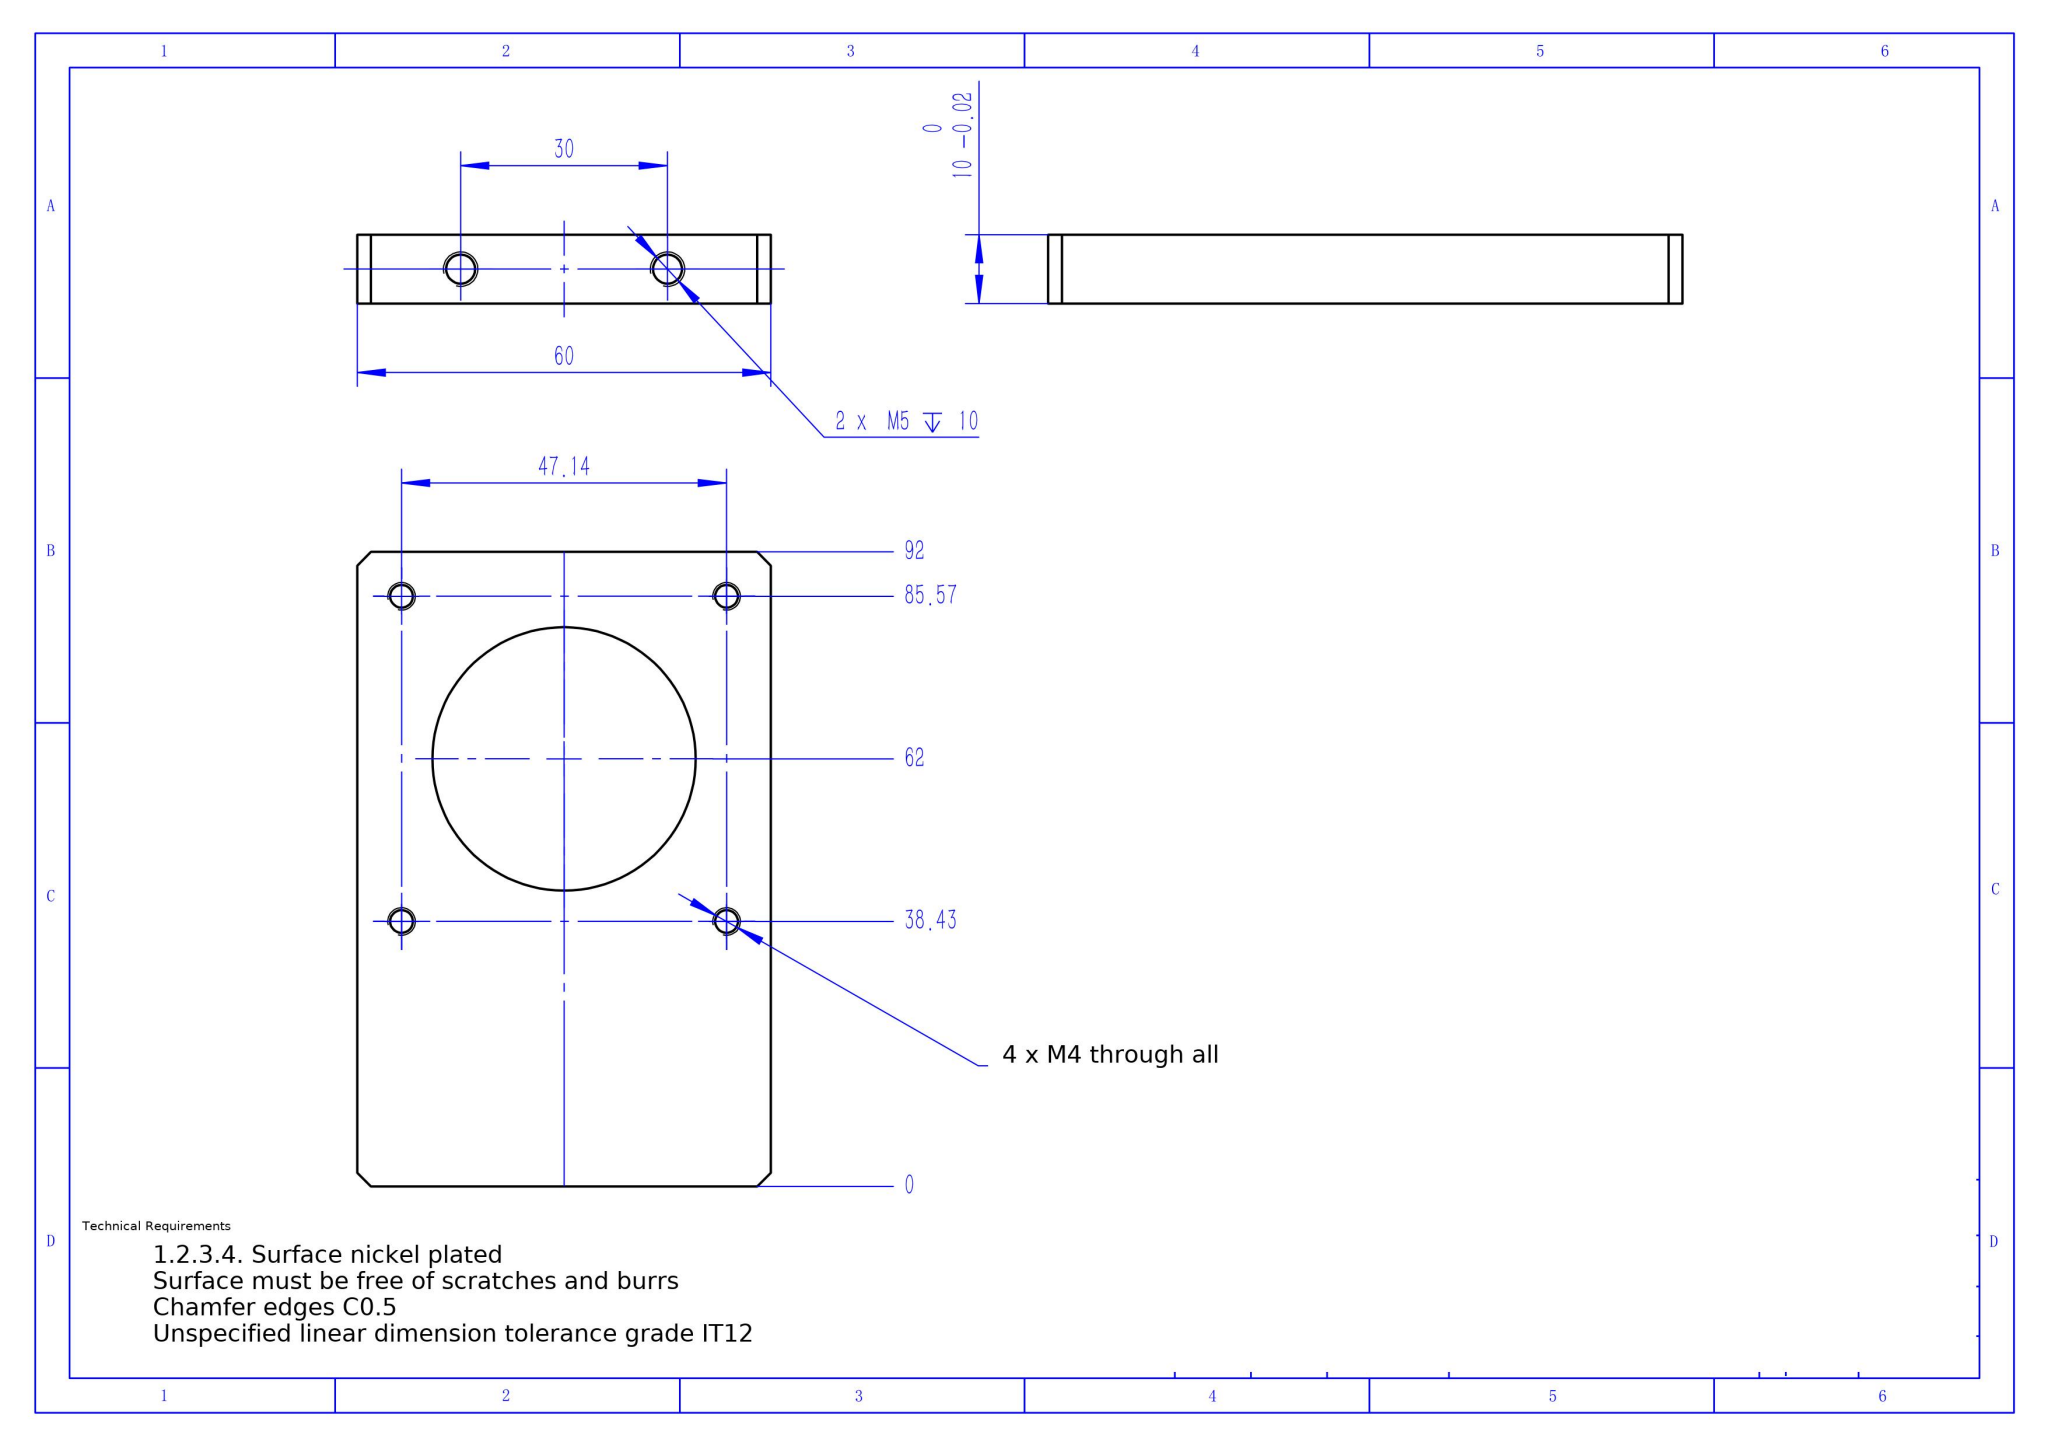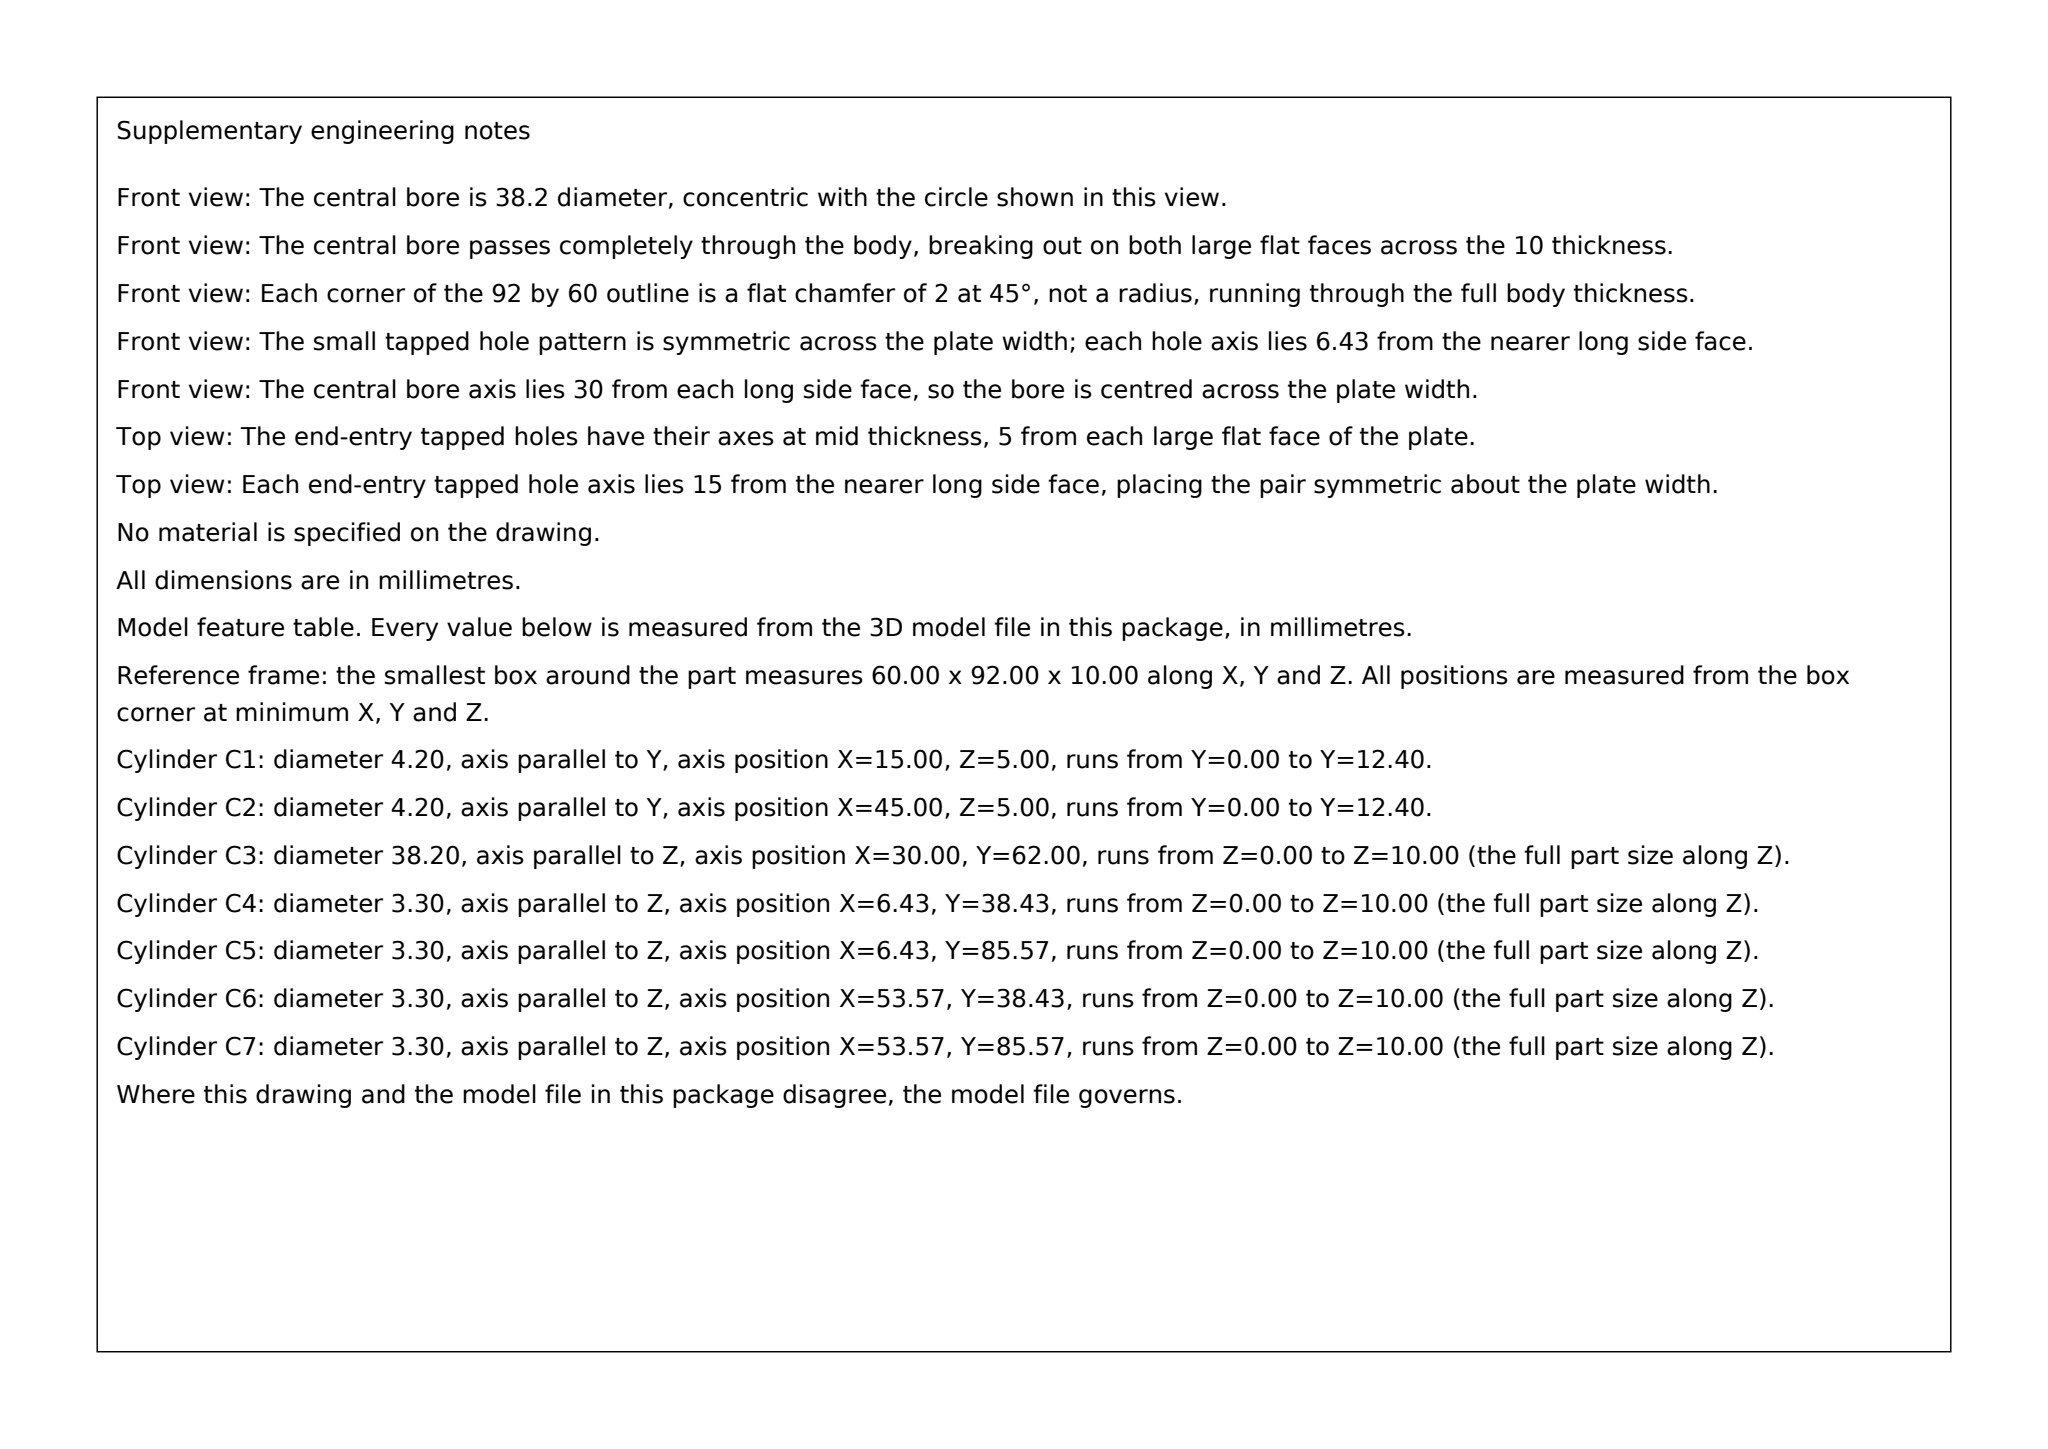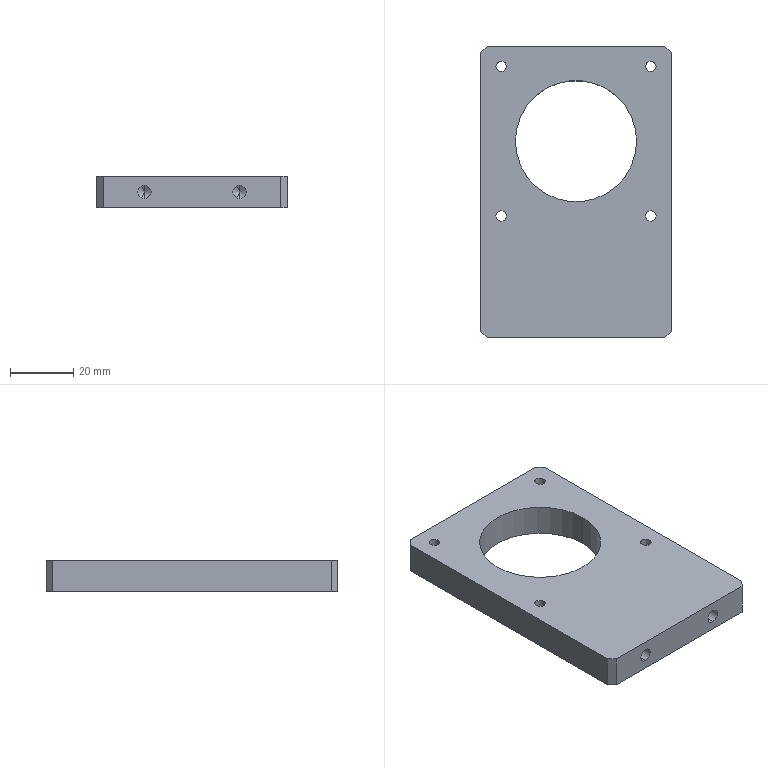Part | SolidWorks | mm | 1 solid | 28 faces | box 60 x 92 x 10 mm | volume 42962 mm3 | cylinder 14 | plane 10 | cone 4 | commonest cylinder face diameters 3.3 x8 4.2 x4 38.2 x2
Drawing notes:
Ø38.2 BORE THRU ALL (10 THK) | from the solid: cylinder dia 38.2, axis z, pos [30.0,62.0], length 10.0 = plate thickness (z planes 0 and 10)
FRONT VIEW OUTLINE 60 X 92, SQUARE CORNERS - NO CORNER RAD | from the solid: Planes x=0/60, y=0/92 only; fillet_radii empty, no corner cylinders
build123d program:
from build123d import *

# Parameters (mm, degrees)
SKETCH1_W             = 60
SKETCH1_H             = 92
SKETCH1_R             = 19.1
BOSS_EXTRUDE1_DEPTH   = 5
M4_TAPPED_HOLE1_D     = 3.3
CHAMFER1_SIZE         = 2
M5_TAPPED_HOLE1_D     = 4.2
M5_TAPPED_HOLE1_DEPTH = 12.4
M5_TAPPED_HOLE1_TIP   = 1.262


with BuildPart() as part:
    # Sketch1 → Boss-Extrude1 (new, symmetric)
    with BuildSketch(Plane.XY):
        with Locations((0, -16)):
            Rectangle(SKETCH1_W, SKETCH1_H)
        Circle(SKETCH1_R, mode=Mode.SUBTRACT)
    extrude(amount=BOSS_EXTRUDE1_DEPTH, both=True)

    # M4 Tapped Hole1 (through all)
    with Locations(Plane(origin=(0, 0, -5), x_dir=(-1, 0, 0), z_dir=(0, 0, -1))):
        with Locations((-23.57, 23.57), (23.57, -23.57), (-23.57, -23.57), (23.57, 23.57)):
            Hole(M4_TAPPED_HOLE1_D / 2)

    # Chamfer1
    chamfer1_edges = [part.edges().sort_by_distance(p)[0] for p in [
        (-30, 30, 0),
        (30, 30, 0),
        (30, -62, 0),
        (-30, -62, 0),
    ]]
    chamfer(chamfer1_edges, length=CHAMFER1_SIZE)

    # M5 Tapped Hole1
    with Locations(Plane(origin=(0, -62, 0), x_dir=(-1, 0, 0), z_dir=(0, -1, 0))):
        with Locations((-15, 0), (15, 0)):
            Hole(M5_TAPPED_HOLE1_D / 2, depth=M5_TAPPED_HOLE1_DEPTH)
            with Locations((0, 0, -(M5_TAPPED_HOLE1_DEPTH + M5_TAPPED_HOLE1_TIP / 2))):  # 118° drill point
                Cone(0, M5_TAPPED_HOLE1_D / 2, M5_TAPPED_HOLE1_TIP, mode=Mode.SUBTRACT)


solid = part.part
STEP:
#1=CARTESIAN_POINT('',(15.,-49.6,2.1));
#2=VERTEX_POINT('',#1);
#3=CARTESIAN_POINT('',(15.,-49.6,-2.1));
#4=VERTEX_POINT('',#3);
#5=CARTESIAN_POINT('',(15.,-49.6,0.));
#6=DIRECTION('',(0.,-1.,0.));
#7=DIRECTION('',(0.,0.,-1.));
#8=AXIS2_PLACEMENT_3D('',#5,#6,#7);
#9=CIRCLE('',#8,2.1);
#10=EDGE_CURVE('',#2,#4,#9,.T.);
#11=ORIENTED_EDGE('',*,*,#10,.F.);
#12=CARTESIAN_POINT('',(15.,-62.,2.1));
#13=VERTEX_POINT('',#12);
#14=CARTESIAN_POINT('',(15.,-62.,2.1));
#15=DIRECTION('',(0.,-1.,0.));
#16=VECTOR('',#15,1000.);
#17=LINE('',#14,#16);
#18=EDGE_CURVE('',#2,#13,#17,.T.);
#19=ORIENTED_EDGE('',*,*,#18,.T.);
#20=CARTESIAN_POINT('',(15.,-62.,-2.1));
#21=VERTEX_POINT('',#20);
#22=CARTESIAN_POINT('',(15.,-62.,0.));
#23=DIRECTION('',(0.,-1.,0.));
#24=DIRECTION('',(0.,0.,-1.));
#25=AXIS2_PLACEMENT_3D('',#22,#23,#24);
#26=CIRCLE('',#25,2.1);
#27=EDGE_CURVE('',#13,#21,#26,.T.);
#28=ORIENTED_EDGE('',*,*,#27,.T.);
#29=CARTESIAN_POINT('',(15.,-62.,-2.1));
#30=DIRECTION('',(0.,-1.,0.));
#31=VECTOR('',#30,1000.);
#32=LINE('',#29,#31);
#33=EDGE_CURVE('',#4,#21,#32,.T.);
#34=ORIENTED_EDGE('',*,*,#33,.F.);
#35=EDGE_LOOP('',(#11,#19,#28,#34));
#36=FACE_OUTER_BOUND('',#35,.T.);
#37=CARTESIAN_POINT('',(15.,-62.,0.));
#38=DIRECTION('',(0.,-1.,0.));
#39=DIRECTION('',(0.,0.,-1.));
#40=AXIS2_PLACEMENT_3D('',#37,#38,#39);
#41=CYLINDRICAL_SURFACE('',#40,2.1);
#42=ADVANCED_FACE('',(#36),#41,.F.);
#43=CARTESIAN_POINT('',(15.,-48.338,0.));
#44=VERTEX_POINT('',#43);
#45=CARTESIAN_POINT('',(15.,-49.6,-2.1));
#46=DIRECTION('',(0.,-0.515,-0.8572));
#47=VECTOR('',#46,1000.);
#48=LINE('',#45,#47);
#49=EDGE_CURVE('',#44,#4,#48,.T.);
#50=ORIENTED_EDGE('',*,*,#49,.F.);
#51=CARTESIAN_POINT('',(15.,-49.6,2.1));
#52=DIRECTION('',(0.,-0.515,0.8572));
#53=VECTOR('',#52,1000.);
#54=LINE('',#51,#53);
#55=EDGE_CURVE('',#44,#2,#54,.T.);
#56=ORIENTED_EDGE('',*,*,#55,.T.);
#57=ORIENTED_EDGE('',*,*,#10,.T.);
#58=EDGE_LOOP('',(#50,#56,#57));
#59=FACE_OUTER_BOUND('',#58,.T.);
#60=CARTESIAN_POINT('',(15.,-49.6,0.));
#61=DIRECTION('',(0.,-1.,0.));
#62=DIRECTION('',(0.,0.,-1.));
#63=AXIS2_PLACEMENT_3D('',#60,#61,#62);
#64=CONICAL_SURFACE('',#63,2.1,1.03);
#65=ADVANCED_FACE('',(#59),#64,.F.);
#66=CARTESIAN_POINT('',(-15.,-49.6,2.1));
#67=VERTEX_POINT('',#66);
#68=CARTESIAN_POINT('',(-15.,-49.6,-2.1));
#69=VERTEX_POINT('',#68);
#70=CARTESIAN_POINT('',(-15.,-49.6,0.));
#71=DIRECTION('',(0.,-1.,0.));
#72=DIRECTION('',(0.,0.,-1.));
#73=AXIS2_PLACEMENT_3D('',#70,#71,#72);
#74=CIRCLE('',#73,2.1);
#75=EDGE_CURVE('',#67,#69,#74,.T.);
#76=ORIENTED_EDGE('',*,*,#75,.F.);
#77=CARTESIAN_POINT('',(-15.,-62.,2.1));
#78=VERTEX_POINT('',#77);
#79=CARTESIAN_POINT('',(-15.,-62.,2.1));
#80=DIRECTION('',(0.,-1.,0.));
#81=VECTOR('',#80,1000.);
#82=LINE('',#79,#81);
#83=EDGE_CURVE('',#67,#78,#82,.T.);
#84=ORIENTED_EDGE('',*,*,#83,.T.);
#85=CARTESIAN_POINT('',(-15.,-62.,-2.1));
#86=VERTEX_POINT('',#85);
#87=CARTESIAN_POINT('',(-15.,-62.,0.));
#88=DIRECTION('',(0.,-1.,0.));
#89=DIRECTION('',(0.,0.,-1.));
#90=AXIS2_PLACEMENT_3D('',#87,#88,#89);
#91=CIRCLE('',#90,2.1);
#92=EDGE_CURVE('',#78,#86,#91,.T.);
#93=ORIENTED_EDGE('',*,*,#92,.T.);
#94=CARTESIAN_POINT('',(-15.,-62.,-2.1));
#95=DIRECTION('',(0.,-1.,0.));
#96=VECTOR('',#95,1000.);
#97=LINE('',#94,#96);
#98=EDGE_CURVE('',#69,#86,#97,.T.);
#99=ORIENTED_EDGE('',*,*,#98,.F.);
#100=EDGE_LOOP('',(#76,#84,#93,#99));
#101=FACE_OUTER_BOUND('',#100,.T.);
#102=CARTESIAN_POINT('',(-15.,-62.,0.));
#103=DIRECTION('',(0.,-1.,0.));
#104=DIRECTION('',(0.,0.,-1.));
#105=AXIS2_PLACEMENT_3D('',#102,#103,#104);
#106=CYLINDRICAL_SURFACE('',#105,2.1);
#107=ADVANCED_FACE('',(#101),#106,.F.);
#108=CARTESIAN_POINT('',(-15.,-48.338,0.));
#109=VERTEX_POINT('',#108);
#110=CARTESIAN_POINT('',(-15.,-49.6,-2.1));
#111=DIRECTION('',(0.,-0.515,-0.8572));
#112=VECTOR('',#111,1000.);
#113=LINE('',#110,#112);
#114=EDGE_CURVE('',#109,#69,#113,.T.);
#115=ORIENTED_EDGE('',*,*,#114,.F.);
#116=CARTESIAN_POINT('',(-15.,-49.6,2.1));
#117=DIRECTION('',(0.,-0.515,0.8572));
#118=VECTOR('',#117,1000.);
#119=LINE('',#116,#118);
#120=EDGE_CURVE('',#109,#67,#119,.T.);
#121=ORIENTED_EDGE('',*,*,#120,.T.);
#122=ORIENTED_EDGE('',*,*,#75,.T.);
#123=EDGE_LOOP('',(#115,#121,#122));
#124=FACE_OUTER_BOUND('',#123,.T.);
#125=CARTESIAN_POINT('',(-15.,-49.6,0.));
#126=DIRECTION('',(0.,-1.,0.));
#127=DIRECTION('',(0.,0.,-1.));
#128=AXIS2_PLACEMENT_3D('',#125,#126,#127);
#129=CONICAL_SURFACE('',#128,2.1,1.03);
#130=ADVANCED_FACE('',(#124),#129,.F.);
#131=CARTESIAN_POINT('',(25.22,23.57,5.));
#132=VERTEX_POINT('',#131);
#133=CARTESIAN_POINT('',(21.92,23.57,5.));
#134=VERTEX_POINT('',#133);
#135=CARTESIAN_POINT('',(23.57,23.57,5.));
#136=DIRECTION('',(0.,0.,-1.));
#137=DIRECTION('',(-1.,0.,0.));
#138=AXIS2_PLACEMENT_3D('',#135,#136,#137);
#139=CIRCLE('',#138,1.65);
#140=EDGE_CURVE('',#132,#134,#139,.T.);
#141=ORIENTED_EDGE('',*,*,#140,.F.);
#142=CARTESIAN_POINT('',(25.22,23.57,-5.));
#143=VERTEX_POINT('',#142);
#144=CARTESIAN_POINT('',(25.22,23.57,-5.));
#145=DIRECTION('',(0.,0.,-1.));
#146=VECTOR('',#145,1000.);
#147=LINE('',#144,#146);
#148=EDGE_CURVE('',#132,#143,#147,.T.);
#149=ORIENTED_EDGE('',*,*,#148,.T.);
#150=CARTESIAN_POINT('',(21.92,23.57,-5.));
#151=VERTEX_POINT('',#150);
#152=CARTESIAN_POINT('',(23.57,23.57,-5.));
#153=DIRECTION('',(0.,0.,-1.));
#154=DIRECTION('',(-1.,0.,0.));
#155=AXIS2_PLACEMENT_3D('',#152,#153,#154);
#156=CIRCLE('',#155,1.65);
#157=EDGE_CURVE('',#143,#151,#156,.T.);
#158=ORIENTED_EDGE('',*,*,#157,.T.);
#159=CARTESIAN_POINT('',(21.92,23.57,-5.));
#160=DIRECTION('',(0.,0.,-1.));
#161=VECTOR('',#160,1000.);
#162=LINE('',#159,#161);
#163=EDGE_CURVE('',#134,#151,#162,.T.);
#164=ORIENTED_EDGE('',*,*,#163,.F.);
#165=EDGE_LOOP('',(#141,#149,#158,#164));
#166=FACE_OUTER_BOUND('',#165,.T.);
#167=CARTESIAN_POINT('',(23.57,23.57,-5.));
#168=DIRECTION('',(0.,0.,-1.));
#169=DIRECTION('',(-1.,0.,0.));
#170=AXIS2_PLACEMENT_3D('',#167,#168,#169);
#171=CYLINDRICAL_SURFACE('',#170,1.65);
#172=ADVANCED_FACE('',(#166),#171,.F.);
#173=CARTESIAN_POINT('',(-21.92,-23.57,5.));
#174=VERTEX_POINT('',#173);
#175=CARTESIAN_POINT('',(-25.22,-23.57,5.));
#176=VERTEX_POINT('',#175);
#177=CARTESIAN_POINT('',(-23.57,-23.57,5.));
#178=DIRECTION('',(0.,0.,-1.));
#179=DIRECTION('',(-1.,0.,0.));
#180=AXIS2_PLACEMENT_3D('',#177,#178,#179);
#181=CIRCLE('',#180,1.65);
#182=EDGE_CURVE('',#174,#176,#181,.T.);
#183=ORIENTED_EDGE('',*,*,#182,.F.);
#184=CARTESIAN_POINT('',(-21.92,-23.57,-5.));
#185=VERTEX_POINT('',#184);
#186=CARTESIAN_POINT('',(-21.92,-23.57,-5.));
#187=DIRECTION('',(0.,0.,-1.));
#188=VECTOR('',#187,1000.);
#189=LINE('',#186,#188);
#190=EDGE_CURVE('',#174,#185,#189,.T.);
#191=ORIENTED_EDGE('',*,*,#190,.T.);
#192=CARTESIAN_POINT('',(-25.22,-23.57,-5.));
#193=VERTEX_POINT('',#192);
#194=CARTESIAN_POINT('',(-23.57,-23.57,-5.));
#195=DIRECTION('',(0.,0.,-1.));
#196=DIRECTION('',(-1.,0.,0.));
#197=AXIS2_PLACEMENT_3D('',#194,#195,#196);
#198=CIRCLE('',#197,1.65);
#199=EDGE_CURVE('',#185,#193,#198,.T.);
#200=ORIENTED_EDGE('',*,*,#199,.T.);
#201=CARTESIAN_POINT('',(-25.22,-23.57,-5.));
#202=DIRECTION('',(0.,0.,-1.));
#203=VECTOR('',#202,1000.);
#204=LINE('',#201,#203);
#205=EDGE_CURVE('',#176,#193,#204,.T.);
#206=ORIENTED_EDGE('',*,*,#205,.F.);
#207=EDGE_LOOP('',(#183,#191,#200,#206));
#208=FACE_OUTER_BOUND('',#207,.T.);
#209=CARTESIAN_POINT('',(-23.57,-23.57,-5.));
#210=DIRECTION('',(0.,0.,-1.));
#211=DIRECTION('',(-1.,0.,0.));
#212=AXIS2_PLACEMENT_3D('',#209,#210,#211);
#213=CYLINDRICAL_SURFACE('',#212,1.65);
#214=ADVANCED_FACE('',(#208),#213,.F.);
#215=CARTESIAN_POINT('',(25.22,-23.57,5.));
#216=VERTEX_POINT('',#215);
#217=CARTESIAN_POINT('',(21.92,-23.57,5.));
#218=VERTEX_POINT('',#217);
#219=CARTESIAN_POINT('',(23.57,-23.57,5.));
#220=DIRECTION('',(0.,0.,-1.));
#221=DIRECTION('',(-1.,0.,0.));
#222=AXIS2_PLACEMENT_3D('',#219,#220,#221);
#223=CIRCLE('',#222,1.65);
#224=EDGE_CURVE('',#216,#218,#223,.T.);
#225=ORIENTED_EDGE('',*,*,#224,.F.);
#226=CARTESIAN_POINT('',(25.22,-23.57,-5.));
#227=VERTEX_POINT('',#226);
#228=CARTESIAN_POINT('',(25.22,-23.57,-5.));
#229=DIRECTION('',(0.,0.,-1.));
#230=VECTOR('',#229,1000.);
#231=LINE('',#228,#230);
#232=EDGE_CURVE('',#216,#227,#231,.T.);
#233=ORIENTED_EDGE('',*,*,#232,.T.);
#234=CARTESIAN_POINT('',(21.92,-23.57,-5.));
#235=VERTEX_POINT('',#234);
#236=CARTESIAN_POINT('',(23.57,-23.57,-5.));
#237=DIRECTION('',(0.,0.,-1.));
#238=DIRECTION('',(-1.,0.,0.));
#239=AXIS2_PLACEMENT_3D('',#236,#237,#238);
#240=CIRCLE('',#239,1.65);
#241=EDGE_CURVE('',#227,#235,#240,.T.);
#242=ORIENTED_EDGE('',*,*,#241,.T.);
#243=CARTESIAN_POINT('',(21.92,-23.57,-5.));
#244=DIRECTION('',(0.,0.,-1.));
#245=VECTOR('',#244,1000.);
#246=LINE('',#243,#245);
#247=EDGE_CURVE('',#218,#235,#246,.T.);
#248=ORIENTED_EDGE('',*,*,#247,.F.);
#249=EDGE_LOOP('',(#225,#233,#242,#248));
#250=FACE_OUTER_BOUND('',#249,.T.);
#251=CARTESIAN_POINT('',(23.57,-23.57,-5.));
#252=DIRECTION('',(0.,0.,-1.));
#253=DIRECTION('',(-1.,0.,0.));
#254=AXIS2_PLACEMENT_3D('',#251,#252,#253);
#255=CYLINDRICAL_SURFACE('',#254,1.65);
#256=ADVANCED_FACE('',(#250),#255,.F.);
#257=CARTESIAN_POINT('',(-21.92,23.57,5.));
#258=VERTEX_POINT('',#257);
#259=CARTESIAN_POINT('',(-25.22,23.57,5.));
#260=VERTEX_POINT('',#259);
#261=CARTESIAN_POINT('',(-23.57,23.57,5.));
#262=DIRECTION('',(0.,0.,-1.));
#263=DIRECTION('',(-1.,0.,0.));
#264=AXIS2_PLACEMENT_3D('',#261,#262,#263);
#265=CIRCLE('',#264,1.65);
#266=EDGE_CURVE('',#258,#260,#265,.T.);
#267=ORIENTED_EDGE('',*,*,#266,.F.);
#268=CARTESIAN_POINT('',(-21.92,23.57,-5.));
#269=VERTEX_POINT('',#268);
#270=CARTESIAN_POINT('',(-21.92,23.57,-5.));
#271=DIRECTION('',(0.,0.,-1.));
#272=VECTOR('',#271,1000.);
#273=LINE('',#270,#272);
#274=EDGE_CURVE('',#258,#269,#273,.T.);
#275=ORIENTED_EDGE('',*,*,#274,.T.);
#276=CARTESIAN_POINT('',(-25.22,23.57,-5.));
#277=VERTEX_POINT('',#276);
#278=CARTESIAN_POINT('',(-23.57,23.57,-5.));
#279=DIRECTION('',(0.,0.,-1.));
#280=DIRECTION('',(-1.,0.,0.));
#281=AXIS2_PLACEMENT_3D('',#278,#279,#280);
#282=CIRCLE('',#281,1.65);
#283=EDGE_CURVE('',#269,#277,#282,.T.);
#284=ORIENTED_EDGE('',*,*,#283,.T.);
#285=CARTESIAN_POINT('',(-25.22,23.57,-5.));
#286=DIRECTION('',(0.,0.,-1.));
#287=VECTOR('',#286,1000.);
#288=LINE('',#285,#287);
#289=EDGE_CURVE('',#260,#277,#288,.T.);
#290=ORIENTED_EDGE('',*,*,#289,.F.);
#291=EDGE_LOOP('',(#267,#275,#284,#290));
#292=FACE_OUTER_BOUND('',#291,.T.);
#293=CARTESIAN_POINT('',(-23.57,23.57,-5.));
#294=DIRECTION('',(0.,0.,-1.));
#295=DIRECTION('',(-1.,0.,0.));
#296=AXIS2_PLACEMENT_3D('',#293,#294,#295);
#297=CYLINDRICAL_SURFACE('',#296,1.65);
#298=ADVANCED_FACE('',(#292),#297,.F.);
#299=CARTESIAN_POINT('',(-19.1,0.,-5.));
#300=VERTEX_POINT('',#299);
#301=CARTESIAN_POINT('',(19.1,0.,-5.));
#302=VERTEX_POINT('',#301);
#303=CARTESIAN_POINT('',(0.,0.,-5.));
#304=DIRECTION('',(0.,0.,1.));
#305=DIRECTION('',(1.,0.,0.));
#306=AXIS2_PLACEMENT_3D('',#303,#304,#305);
#307=CIRCLE('',#306,19.1);
#308=EDGE_CURVE('',#300,#302,#307,.T.);
#309=ORIENTED_EDGE('',*,*,#308,.F.);
#310=CARTESIAN_POINT('',(-19.1,0.,5.));
#311=VERTEX_POINT('',#310);
#312=CARTESIAN_POINT('',(-19.1,0.,-5.));
#313=DIRECTION('',(0.,0.,1.));
#314=VECTOR('',#313,1000.);
#315=LINE('',#312,#314);
#316=EDGE_CURVE('',#300,#311,#315,.T.);
#317=ORIENTED_EDGE('',*,*,#316,.T.);
#318=CARTESIAN_POINT('',(19.1,0.,5.));
#319=VERTEX_POINT('',#318);
#320=CARTESIAN_POINT('',(0.,0.,5.));
#321=DIRECTION('',(0.,0.,1.));
#322=DIRECTION('',(1.,0.,0.));
#323=AXIS2_PLACEMENT_3D('',#320,#321,#322);
#324=CIRCLE('',#323,19.1);
#325=EDGE_CURVE('',#311,#319,#324,.T.);
#326=ORIENTED_EDGE('',*,*,#325,.T.);
#327=CARTESIAN_POINT('',(19.1,0.,-5.));
#328=DIRECTION('',(0.,0.,1.));
#329=VECTOR('',#328,1000.);
#330=LINE('',#327,#329);
#331=EDGE_CURVE('',#302,#319,#330,.T.);
#332=ORIENTED_EDGE('',*,*,#331,.F.);
#333=EDGE_LOOP('',(#309,#317,#326,#332));
#334=FACE_OUTER_BOUND('',#333,.T.);
#335=CARTESIAN_POINT('',(0.,0.,-5.));
#336=DIRECTION('',(0.,0.,1.));
#337=DIRECTION('',(1.,0.,0.));
#338=AXIS2_PLACEMENT_3D('',#335,#336,#337);
#339=CYLINDRICAL_SURFACE('',#338,19.1);
#340=ADVANCED_FACE('',(#334),#339,.F.);
#341=CARTESIAN_POINT('',(-30.,28.,-5.));
#342=VERTEX_POINT('',#341);
#343=CARTESIAN_POINT('',(-30.,-60.,-5.));
#344=VERTEX_POINT('',#343);
#345=CARTESIAN_POINT('',(-30.,30.,-5.));
#346=DIRECTION('',(-0.,-1.,0.));
#347=VECTOR('',#346,1000.);
#348=LINE('',#345,#347);
#349=EDGE_CURVE('',#342,#344,#348,.T.);
#350=ORIENTED_EDGE('',*,*,#349,.T.);
#351=CARTESIAN_POINT('',(-30.,-60.,5.));
#352=VERTEX_POINT('',#351);
#353=CARTESIAN_POINT('',(-30.,-60.,-5.));
#354=DIRECTION('',(0.,0.,1.));
#355=VECTOR('',#354,1000.);
#356=LINE('',#353,#355);
#357=EDGE_CURVE('',#344,#352,#356,.T.);
#358=ORIENTED_EDGE('',*,*,#357,.T.);
#359=CARTESIAN_POINT('',(-30.,28.,5.));
#360=VERTEX_POINT('',#359);
#361=CARTESIAN_POINT('',(-30.,30.,5.));
#362=DIRECTION('',(-0.,-1.,0.));
#363=VECTOR('',#362,1000.);
#364=LINE('',#361,#363);
#365=EDGE_CURVE('',#360,#352,#364,.T.);
#366=ORIENTED_EDGE('',*,*,#365,.F.);
#367=CARTESIAN_POINT('',(-30.,28.,-5.));
#368=DIRECTION('',(0.,0.,-1.));
#369=VECTOR('',#368,1000.);
#370=LINE('',#367,#369);
#371=EDGE_CURVE('',#360,#342,#370,.T.);
#372=ORIENTED_EDGE('',*,*,#371,.T.);
#373=EDGE_LOOP('',(#350,#358,#366,#372));
#374=FACE_OUTER_BOUND('',#373,.T.);
#375=CARTESIAN_POINT('',(-30.,30.,-5.));
#376=DIRECTION('',(-1.,0.,0.));
#377=DIRECTION('',(-0.,-1.,0.));
#378=AXIS2_PLACEMENT_3D('',#375,#376,#377);
#379=PLANE('',#378);
#380=ADVANCED_FACE('',(#374),#379,.T.);
#381=CARTESIAN_POINT('',(28.,30.,-5.));
#382=VERTEX_POINT('',#381);
#383=CARTESIAN_POINT('',(-28.,30.,-5.));
#384=VERTEX_POINT('',#383);
#385=CARTESIAN_POINT('',(-30.,30.,-5.));
#386=DIRECTION('',(-1.,0.,0.));
#387=VECTOR('',#386,1000.);
#388=LINE('',#385,#387);
#389=EDGE_CURVE('',#382,#384,#388,.T.);
#390=ORIENTED_EDGE('',*,*,#389,.T.);
#391=CARTESIAN_POINT('',(-28.,30.,5.));
#392=VERTEX_POINT('',#391);
#393=CARTESIAN_POINT('',(-28.,30.,-5.));
#394=DIRECTION('',(0.,0.,1.));
#395=VECTOR('',#394,1000.);
#396=LINE('',#393,#395);
#397=EDGE_CURVE('',#384,#392,#396,.T.);
#398=ORIENTED_EDGE('',*,*,#397,.T.);
#399=CARTESIAN_POINT('',(28.,30.,5.));
#400=VERTEX_POINT('',#399);
#401=CARTESIAN_POINT('',(-30.,30.,5.));
#402=DIRECTION('',(-1.,0.,0.));
#403=VECTOR('',#402,1000.);
#404=LINE('',#401,#403);
#405=EDGE_CURVE('',#400,#392,#404,.T.);
#406=ORIENTED_EDGE('',*,*,#405,.F.);
#407=CARTESIAN_POINT('',(28.,30.,-5.));
#408=DIRECTION('',(0.,0.,-1.));
#409=VECTOR('',#408,1000.);
#410=LINE('',#407,#409);
#411=EDGE_CURVE('',#400,#382,#410,.T.);
#412=ORIENTED_EDGE('',*,*,#411,.T.);
#413=EDGE_LOOP('',(#390,#398,#406,#412));
#414=FACE_OUTER_BOUND('',#413,.T.);
#415=CARTESIAN_POINT('',(-30.,30.,-5.));
#416=DIRECTION('',(0.,1.,0.));
#417=DIRECTION('',(0.,0.,1.));
#418=AXIS2_PLACEMENT_3D('',#415,#416,#417);
#419=PLANE('',#418);
#420=ADVANCED_FACE('',(#414),#419,.T.);
#421=CARTESIAN_POINT('',(30.,-60.,5.));
#422=VERTEX_POINT('',#421);
#423=CARTESIAN_POINT('',(30.,28.,5.));
#424=VERTEX_POINT('',#423);
#425=CARTESIAN_POINT('',(30.,30.,5.));
#426=DIRECTION('',(-0.,1.,0.));
#427=VECTOR('',#426,1000.);
#428=LINE('',#425,#427);
#429=EDGE_CURVE('',#422,#424,#428,.T.);
#430=ORIENTED_EDGE('',*,*,#429,.F.);
#431=CARTESIAN_POINT('',(30.,-60.,-5.));
#432=VERTEX_POINT('',#431);
#433=CARTESIAN_POINT('',(30.,-60.,-5.));
#434=DIRECTION('',(0.,0.,-1.));
#435=VECTOR('',#434,1000.);
#436=LINE('',#433,#435);
#437=EDGE_CURVE('',#422,#432,#436,.T.);
#438=ORIENTED_EDGE('',*,*,#437,.T.);
#439=CARTESIAN_POINT('',(30.,28.,-5.));
#440=VERTEX_POINT('',#439);
#441=CARTESIAN_POINT('',(30.,30.,-5.));
#442=DIRECTION('',(-0.,1.,0.));
#443=VECTOR('',#442,1000.);
#444=LINE('',#441,#443);
#445=EDGE_CURVE('',#432,#440,#444,.T.);
#446=ORIENTED_EDGE('',*,*,#445,.T.);
#447=CARTESIAN_POINT('',(30.,28.,-5.));
#448=DIRECTION('',(0.,0.,1.));
#449=VECTOR('',#448,1000.);
#450=LINE('',#447,#449);
#451=EDGE_CURVE('',#440,#424,#450,.T.);
#452=ORIENTED_EDGE('',*,*,#451,.T.);
#453=EDGE_LOOP('',(#430,#438,#446,#452));
#454=FACE_OUTER_BOUND('',#453,.T.);
#455=CARTESIAN_POINT('',(30.,30.,-5.));
#456=DIRECTION('',(1.,0.,0.));
#457=DIRECTION('',(-0.,1.,0.));
#458=AXIS2_PLACEMENT_3D('',#455,#456,#457);
#459=PLANE('',#458);
#460=ADVANCED_FACE('',(#454),#459,.T.);
#461=CARTESIAN_POINT('',(15.,-62.,0.));
#462=DIRECTION('',(0.,-1.,0.));
#463=DIRECTION('',(0.,0.,-1.));
#464=AXIS2_PLACEMENT_3D('',#461,#462,#463);
#465=CIRCLE('',#464,2.1);
#466=EDGE_CURVE('',#21,#13,#465,.T.);
#467=ORIENTED_EDGE('',*,*,#466,.F.);
#468=ORIENTED_EDGE('',*,*,#27,.F.);
#469=EDGE_LOOP('',(#467,#468));
#470=FACE_BOUND('',#469,.T.);
#471=CARTESIAN_POINT('',(-15.,-62.,0.));
#472=DIRECTION('',(0.,-1.,0.));
#473=DIRECTION('',(0.,0.,-1.));
#474=AXIS2_PLACEMENT_3D('',#471,#472,#473);
#475=CIRCLE('',#474,2.1);
#476=EDGE_CURVE('',#86,#78,#475,.T.);
#477=ORIENTED_EDGE('',*,*,#476,.F.);
#478=ORIENTED_EDGE('',*,*,#92,.F.);
#479=EDGE_LOOP('',(#477,#478));
#480=FACE_BOUND('',#479,.T.);
#481=CARTESIAN_POINT('',(-28.,-62.,5.));
#482=VERTEX_POINT('',#481);
#483=CARTESIAN_POINT('',(28.,-62.,5.));
#484=VERTEX_POINT('',#483);
#485=CARTESIAN_POINT('',(-30.,-62.,5.));
#486=DIRECTION('',(1.,0.,0.));
#487=VECTOR('',#486,1000.);
#488=LINE('',#485,#487);
#489=EDGE_CURVE('',#482,#484,#488,.T.);
#490=ORIENTED_EDGE('',*,*,#489,.F.);
#491=CARTESIAN_POINT('',(-28.,-62.,-5.));
#492=VERTEX_POINT('',#491);
#493=CARTESIAN_POINT('',(-28.,-62.,-5.));
#494=DIRECTION('',(0.,0.,-1.));
#495=VECTOR('',#494,1000.);
#496=LINE('',#493,#495);
#497=EDGE_CURVE('',#482,#492,#496,.T.);
#498=ORIENTED_EDGE('',*,*,#497,.T.);
#499=CARTESIAN_POINT('',(28.,-62.,-5.));
#500=VERTEX_POINT('',#499);
#501=CARTESIAN_POINT('',(-30.,-62.,-5.));
#502=DIRECTION('',(1.,0.,0.));
#503=VECTOR('',#502,1000.);
#504=LINE('',#501,#503);
#505=EDGE_CURVE('',#492,#500,#504,.T.);
#506=ORIENTED_EDGE('',*,*,#505,.T.);
#507=CARTESIAN_POINT('',(28.,-62.,-5.));
#508=DIRECTION('',(0.,0.,1.));
#509=VECTOR('',#508,1000.);
#510=LINE('',#507,#509);
#511=EDGE_CURVE('',#500,#484,#510,.T.);
#512=ORIENTED_EDGE('',*,*,#511,.T.);
#513=EDGE_LOOP('',(#490,#498,#506,#512));
#514=FACE_OUTER_BOUND('',#513,.T.);
#515=CARTESIAN_POINT('',(-30.,-62.,-5.));
#516=DIRECTION('',(0.,-1.,0.));
#517=DIRECTION('',(0.,0.,-1.));
#518=AXIS2_PLACEMENT_3D('',#515,#516,#517);
#519=PLANE('',#518);
#520=ADVANCED_FACE('',(#470,#480,#514),#519,.T.);
#521=CARTESIAN_POINT('',(23.57,23.57,-5.));
#522=DIRECTION('',(0.,0.,-1.));
#523=DIRECTION('',(-1.,0.,0.));
#524=AXIS2_PLACEMENT_3D('',#521,#522,#523);
#525=CIRCLE('',#524,1.65);
#526=EDGE_CURVE('',#151,#143,#525,.T.);
#527=ORIENTED_EDGE('',*,*,#526,.F.);
#528=ORIENTED_EDGE('',*,*,#157,.F.);
#529=EDGE_LOOP('',(#527,#528));
#530=FACE_BOUND('',#529,.T.);
#531=CARTESIAN_POINT('',(-23.57,-23.57,-5.));
#532=DIRECTION('',(0.,0.,-1.));
#533=DIRECTION('',(-1.,0.,0.));
#534=AXIS2_PLACEMENT_3D('',#531,#532,#533);
#535=CIRCLE('',#534,1.65);
#536=EDGE_CURVE('',#193,#185,#535,.T.);
#537=ORIENTED_EDGE('',*,*,#536,.F.);
#538=ORIENTED_EDGE('',*,*,#199,.F.);
#539=EDGE_LOOP('',(#537,#538));
#540=FACE_BOUND('',#539,.T.);
#541=CARTESIAN_POINT('',(23.57,-23.57,-5.));
#542=DIRECTION('',(0.,0.,-1.));
#543=DIRECTION('',(-1.,0.,0.));
#544=AXIS2_PLACEMENT_3D('',#541,#542,#543);
#545=CIRCLE('',#544,1.65);
#546=EDGE_CURVE('',#235,#227,#545,.T.);
#547=ORIENTED_EDGE('',*,*,#546,.F.);
#548=ORIENTED_EDGE('',*,*,#241,.F.);
#549=EDGE_LOOP('',(#547,#548));
#550=FACE_BOUND('',#549,.T.);
#551=CARTESIAN_POINT('',(-23.57,23.57,-5.));
#552=DIRECTION('',(0.,0.,-1.));
#553=DIRECTION('',(-1.,0.,0.));
#554=AXIS2_PLACEMENT_3D('',#551,#552,#553);
#555=CIRCLE('',#554,1.65);
#556=EDGE_CURVE('',#277,#269,#555,.T.);
#557=ORIENTED_EDGE('',*,*,#556,.F.);
#558=ORIENTED_EDGE('',*,*,#283,.F.);
#559=EDGE_LOOP('',(#557,#558));
#560=FACE_BOUND('',#559,.T.);
#561=CARTESIAN_POINT('',(0.,0.,-5.));
#562=DIRECTION('',(0.,0.,1.));
#563=DIRECTION('',(1.,0.,0.));
#564=AXIS2_PLACEMENT_3D('',#561,#562,#563);
#565=CIRCLE('',#564,19.1);
#566=EDGE_CURVE('',#302,#300,#565,.T.);
#567=ORIENTED_EDGE('',*,*,#566,.T.);
#568=ORIENTED_EDGE('',*,*,#308,.T.);
#569=EDGE_LOOP('',(#567,#568));
#570=FACE_BOUND('',#569,.T.);
#571=ORIENTED_EDGE('',*,*,#505,.F.);
#572=CARTESIAN_POINT('',(-30.,-60.,-5.));
#573=DIRECTION('',(-0.7071,0.7071,0.));
#574=VECTOR('',#573,1000.);
#575=LINE('',#572,#574);
#576=EDGE_CURVE('',#492,#344,#575,.T.);
#577=ORIENTED_EDGE('',*,*,#576,.T.);
#578=ORIENTED_EDGE('',*,*,#349,.F.);
#579=CARTESIAN_POINT('',(-28.,30.,-5.));
#580=DIRECTION('',(0.7071,0.7071,0.));
#581=VECTOR('',#580,1000.);
#582=LINE('',#579,#581);
#583=EDGE_CURVE('',#342,#384,#582,.T.);
#584=ORIENTED_EDGE('',*,*,#583,.T.);
#585=ORIENTED_EDGE('',*,*,#389,.F.);
#586=CARTESIAN_POINT('',(30.,28.,-5.));
#587=DIRECTION('',(0.7071,-0.7071,0.));
#588=VECTOR('',#587,1000.);
#589=LINE('',#586,#588);
#590=EDGE_CURVE('',#382,#440,#589,.T.);
#591=ORIENTED_EDGE('',*,*,#590,.T.);
#592=ORIENTED_EDGE('',*,*,#445,.F.);
#593=CARTESIAN_POINT('',(28.,-62.,-5.));
#594=DIRECTION('',(-0.7071,-0.7071,0.));
#595=VECTOR('',#594,1000.);
#596=LINE('',#593,#595);
#597=EDGE_CURVE('',#432,#500,#596,.T.);
#598=ORIENTED_EDGE('',*,*,#597,.T.);
#599=EDGE_LOOP('',(#571,#577,#578,#584,#585,#591,#592,#598));
#600=FACE_OUTER_BOUND('',#599,.T.);
#601=CARTESIAN_POINT('',(0.,0.,-5.));
#602=DIRECTION('',(0.,0.,1.));
#603=DIRECTION('',(1.,0.,0.));
#604=AXIS2_PLACEMENT_3D('',#601,#602,#603);
#605=PLANE('',#604);
#606=ADVANCED_FACE('',(#530,#540,#550,#560,#570,#600),#605,.F.);
#607=CARTESIAN_POINT('',(23.57,23.57,5.));
#608=DIRECTION('',(0.,0.,-1.));
#609=DIRECTION('',(-1.,0.,0.));
#610=AXIS2_PLACEMENT_3D('',#607,#608,#609);
#611=CIRCLE('',#610,1.65);
#612=EDGE_CURVE('',#134,#132,#611,.T.);
#613=ORIENTED_EDGE('',*,*,#612,.T.);
#614=ORIENTED_EDGE('',*,*,#140,.T.);
#615=EDGE_LOOP('',(#613,#614));
#616=FACE_BOUND('',#615,.T.);
#617=CARTESIAN_POINT('',(-23.57,-23.57,5.));
#618=DIRECTION('',(0.,0.,-1.));
#619=DIRECTION('',(-1.,0.,0.));
#620=AXIS2_PLACEMENT_3D('',#617,#618,#619);
#621=CIRCLE('',#620,1.65);
#622=EDGE_CURVE('',#176,#174,#621,.T.);
#623=ORIENTED_EDGE('',*,*,#622,.T.);
#624=ORIENTED_EDGE('',*,*,#182,.T.);
#625=EDGE_LOOP('',(#623,#624));
#626=FACE_BOUND('',#625,.T.);
#627=CARTESIAN_POINT('',(23.57,-23.57,5.));
#628=DIRECTION('',(0.,0.,-1.));
#629=DIRECTION('',(-1.,0.,0.));
#630=AXIS2_PLACEMENT_3D('',#627,#628,#629);
#631=CIRCLE('',#630,1.65);
#632=EDGE_CURVE('',#218,#216,#631,.T.);
#633=ORIENTED_EDGE('',*,*,#632,.T.);
#634=ORIENTED_EDGE('',*,*,#224,.T.);
#635=EDGE_LOOP('',(#633,#634));
#636=FACE_BOUND('',#635,.T.);
#637=CARTESIAN_POINT('',(-23.57,23.57,5.));
#638=DIRECTION('',(0.,0.,-1.));
#639=DIRECTION('',(-1.,0.,0.));
#640=AXIS2_PLACEMENT_3D('',#637,#638,#639);
#641=CIRCLE('',#640,1.65);
#642=EDGE_CURVE('',#260,#258,#641,.T.);
#643=ORIENTED_EDGE('',*,*,#642,.T.);
#644=ORIENTED_EDGE('',*,*,#266,.T.);
#645=EDGE_LOOP('',(#643,#644));
#646=FACE_BOUND('',#645,.T.);
#647=CARTESIAN_POINT('',(0.,0.,5.));
#648=DIRECTION('',(0.,0.,1.));
#649=DIRECTION('',(1.,0.,0.));
#650=AXIS2_PLACEMENT_3D('',#647,#648,#649);
#651=CIRCLE('',#650,19.1);
#652=EDGE_CURVE('',#319,#311,#651,.T.);
#653=ORIENTED_EDGE('',*,*,#652,.F.);
#654=ORIENTED_EDGE('',*,*,#325,.F.);
#655=EDGE_LOOP('',(#653,#654));
#656=FACE_BOUND('',#655,.T.);
#657=ORIENTED_EDGE('',*,*,#365,.T.);
#658=CARTESIAN_POINT('',(-45.,-45.,5.));
#659=DIRECTION('',(0.7071,-0.7071,0.));
#660=VECTOR('',#659,1000.);
#661=LINE('',#658,#660);
#662=EDGE_CURVE('',#352,#482,#661,.T.);
#663=ORIENTED_EDGE('',*,*,#662,.T.);
#664=ORIENTED_EDGE('',*,*,#489,.T.);
#665=CARTESIAN_POINT('',(45.,-45.,5.));
#666=DIRECTION('',(0.7071,0.7071,0.));
#667=VECTOR('',#666,1000.);
#668=LINE('',#665,#667);
#669=EDGE_CURVE('',#484,#422,#668,.T.);
#670=ORIENTED_EDGE('',*,*,#669,.T.);
#671=ORIENTED_EDGE('',*,*,#429,.T.);
#672=CARTESIAN_POINT('',(29.,29.,5.));
#673=DIRECTION('',(-0.7071,0.7071,0.));
#674=VECTOR('',#673,1000.);
#675=LINE('',#672,#674);
#676=EDGE_CURVE('',#424,#400,#675,.T.);
#677=ORIENTED_EDGE('',*,*,#676,.T.);
#678=ORIENTED_EDGE('',*,*,#405,.T.);
#679=CARTESIAN_POINT('',(-29.,29.,5.));
#680=DIRECTION('',(-0.7071,-0.7071,0.));
#681=VECTOR('',#680,1000.);
#682=LINE('',#679,#681);
#683=EDGE_CURVE('',#392,#360,#682,.T.);
#684=ORIENTED_EDGE('',*,*,#683,.T.);
#685=EDGE_LOOP('',(#657,#663,#664,#670,#671,#677,#678,#684));
#686=FACE_OUTER_BOUND('',#685,.T.);
#687=CARTESIAN_POINT('',(0.,0.,5.));
#688=DIRECTION('',(0.,0.,1.));
#689=DIRECTION('',(1.,0.,0.));
#690=AXIS2_PLACEMENT_3D('',#687,#688,#689);
#691=PLANE('',#690);
#692=ADVANCED_FACE('',(#616,#626,#636,#646,#656,#686),#691,.T.);
#693=ORIENTED_EDGE('',*,*,#316,.F.);
#694=ORIENTED_EDGE('',*,*,#566,.F.);
#695=ORIENTED_EDGE('',*,*,#331,.T.);
#696=ORIENTED_EDGE('',*,*,#652,.T.);
#697=EDGE_LOOP('',(#693,#694,#695,#696));
#698=FACE_OUTER_BOUND('',#697,.T.);
#699=CARTESIAN_POINT('',(0.,0.,-5.));
#700=DIRECTION('',(0.,0.,1.));
#701=DIRECTION('',(1.,0.,0.));
#702=AXIS2_PLACEMENT_3D('',#699,#700,#701);
#703=CYLINDRICAL_SURFACE('',#702,19.1);
#704=ADVANCED_FACE('',(#698),#703,.F.);
#705=ORIENTED_EDGE('',*,*,#274,.F.);
#706=ORIENTED_EDGE('',*,*,#642,.F.);
#707=ORIENTED_EDGE('',*,*,#289,.T.);
#708=ORIENTED_EDGE('',*,*,#556,.T.);
#709=EDGE_LOOP('',(#705,#706,#707,#708));
#710=FACE_OUTER_BOUND('',#709,.T.);
#711=CARTESIAN_POINT('',(-23.57,23.57,-5.));
#712=DIRECTION('',(0.,0.,-1.));
#713=DIRECTION('',(-1.,0.,0.));
#714=AXIS2_PLACEMENT_3D('',#711,#712,#713);
#715=CYLINDRICAL_SURFACE('',#714,1.65);
#716=ADVANCED_FACE('',(#710),#715,.F.);
#717=ORIENTED_EDGE('',*,*,#232,.F.);
#718=ORIENTED_EDGE('',*,*,#632,.F.);
#719=ORIENTED_EDGE('',*,*,#247,.T.);
#720=ORIENTED_EDGE('',*,*,#546,.T.);
#721=EDGE_LOOP('',(#717,#718,#719,#720));
#722=FACE_OUTER_BOUND('',#721,.T.);
#723=CARTESIAN_POINT('',(23.57,-23.57,-5.));
#724=DIRECTION('',(0.,0.,-1.));
#725=DIRECTION('',(-1.,0.,0.));
#726=AXIS2_PLACEMENT_3D('',#723,#724,#725);
#727=CYLINDRICAL_SURFACE('',#726,1.65);
#728=ADVANCED_FACE('',(#722),#727,.F.);
#729=ORIENTED_EDGE('',*,*,#190,.F.);
#730=ORIENTED_EDGE('',*,*,#622,.F.);
#731=ORIENTED_EDGE('',*,*,#205,.T.);
#732=ORIENTED_EDGE('',*,*,#536,.T.);
#733=EDGE_LOOP('',(#729,#730,#731,#732));
#734=FACE_OUTER_BOUND('',#733,.T.);
#735=CARTESIAN_POINT('',(-23.57,-23.57,-5.));
#736=DIRECTION('',(0.,0.,-1.));
#737=DIRECTION('',(-1.,0.,0.));
#738=AXIS2_PLACEMENT_3D('',#735,#736,#737);
#739=CYLINDRICAL_SURFACE('',#738,1.65);
#740=ADVANCED_FACE('',(#734),#739,.F.);
#741=ORIENTED_EDGE('',*,*,#148,.F.);
#742=ORIENTED_EDGE('',*,*,#612,.F.);
#743=ORIENTED_EDGE('',*,*,#163,.T.);
#744=ORIENTED_EDGE('',*,*,#526,.T.);
#745=EDGE_LOOP('',(#741,#742,#743,#744));
#746=FACE_OUTER_BOUND('',#745,.T.);
#747=CARTESIAN_POINT('',(23.57,23.57,-5.));
#748=DIRECTION('',(0.,0.,-1.));
#749=DIRECTION('',(-1.,0.,0.));
#750=AXIS2_PLACEMENT_3D('',#747,#748,#749);
#751=CYLINDRICAL_SURFACE('',#750,1.65);
#752=ADVANCED_FACE('',(#746),#751,.F.);
#753=ORIENTED_EDGE('',*,*,#576,.F.);
#754=ORIENTED_EDGE('',*,*,#497,.F.);
#755=ORIENTED_EDGE('',*,*,#662,.F.);
#756=ORIENTED_EDGE('',*,*,#357,.F.);
#757=EDGE_LOOP('',(#753,#754,#755,#756));
#758=FACE_OUTER_BOUND('',#757,.T.);
#759=CARTESIAN_POINT('',(-30.,-60.,-5.));
#760=DIRECTION('',(0.7071,0.7071,0.));
#761=DIRECTION('',(0.,0.,1.));
#762=AXIS2_PLACEMENT_3D('',#759,#760,#761);
#763=PLANE('',#762);
#764=ADVANCED_FACE('',(#758),#763,.F.);
#765=ORIENTED_EDGE('',*,*,#597,.F.);
#766=ORIENTED_EDGE('',*,*,#437,.F.);
#767=ORIENTED_EDGE('',*,*,#669,.F.);
#768=ORIENTED_EDGE('',*,*,#511,.F.);
#769=EDGE_LOOP('',(#765,#766,#767,#768));
#770=FACE_OUTER_BOUND('',#769,.T.);
#771=CARTESIAN_POINT('',(28.,-62.,-5.));
#772=DIRECTION('',(-0.7071,0.7071,0.));
#773=DIRECTION('',(0.,0.,1.));
#774=AXIS2_PLACEMENT_3D('',#771,#772,#773);
#775=PLANE('',#774);
#776=ADVANCED_FACE('',(#770),#775,.F.);
#777=ORIENTED_EDGE('',*,*,#583,.F.);
#778=ORIENTED_EDGE('',*,*,#371,.F.);
#779=ORIENTED_EDGE('',*,*,#683,.F.);
#780=ORIENTED_EDGE('',*,*,#397,.F.);
#781=EDGE_LOOP('',(#777,#778,#779,#780));
#782=FACE_OUTER_BOUND('',#781,.T.);
#783=CARTESIAN_POINT('',(-28.,30.,-5.));
#784=DIRECTION('',(0.7071,-0.7071,0.));
#785=DIRECTION('',(0.,0.,1.));
#786=AXIS2_PLACEMENT_3D('',#783,#784,#785);
#787=PLANE('',#786);
#788=ADVANCED_FACE('',(#782),#787,.F.);
#789=ORIENTED_EDGE('',*,*,#590,.F.);
#790=ORIENTED_EDGE('',*,*,#411,.F.);
#791=ORIENTED_EDGE('',*,*,#676,.F.);
#792=ORIENTED_EDGE('',*,*,#451,.F.);
#793=EDGE_LOOP('',(#789,#790,#791,#792));
#794=FACE_OUTER_BOUND('',#793,.T.);
#795=CARTESIAN_POINT('',(30.,28.,-5.));
#796=DIRECTION('',(-0.7071,-0.7071,0.));
#797=DIRECTION('',(0.,0.,1.));
#798=AXIS2_PLACEMENT_3D('',#795,#796,#797);
#799=PLANE('',#798);
#800=ADVANCED_FACE('',(#794),#799,.F.);
#801=ORIENTED_EDGE('',*,*,#120,.F.);
#802=ORIENTED_EDGE('',*,*,#114,.T.);
#803=CARTESIAN_POINT('',(-15.,-49.6,0.));
#804=DIRECTION('',(0.,-1.,0.));
#805=DIRECTION('',(0.,0.,-1.));
#806=AXIS2_PLACEMENT_3D('',#803,#804,#805);
#807=CIRCLE('',#806,2.1);
#808=EDGE_CURVE('',#69,#67,#807,.T.);
#809=ORIENTED_EDGE('',*,*,#808,.T.);
#810=EDGE_LOOP('',(#801,#802,#809));
#811=FACE_OUTER_BOUND('',#810,.T.);
#812=CARTESIAN_POINT('',(-15.,-49.6,0.));
#813=DIRECTION('',(0.,-1.,0.));
#814=DIRECTION('',(0.,0.,-1.));
#815=AXIS2_PLACEMENT_3D('',#812,#813,#814);
#816=CONICAL_SURFACE('',#815,2.1,1.03);
#817=ADVANCED_FACE('',(#811),#816,.F.);
#818=ORIENTED_EDGE('',*,*,#83,.F.);
#819=ORIENTED_EDGE('',*,*,#808,.F.);
#820=ORIENTED_EDGE('',*,*,#98,.T.);
#821=ORIENTED_EDGE('',*,*,#476,.T.);
#822=EDGE_LOOP('',(#818,#819,#820,#821));
#823=FACE_OUTER_BOUND('',#822,.T.);
#824=CARTESIAN_POINT('',(-15.,-62.,0.));
#825=DIRECTION('',(0.,-1.,0.));
#826=DIRECTION('',(0.,0.,-1.));
#827=AXIS2_PLACEMENT_3D('',#824,#825,#826);
#828=CYLINDRICAL_SURFACE('',#827,2.1);
#829=ADVANCED_FACE('',(#823),#828,.F.);
#830=ORIENTED_EDGE('',*,*,#55,.F.);
#831=ORIENTED_EDGE('',*,*,#49,.T.);
#832=CARTESIAN_POINT('',(15.,-49.6,0.));
#833=DIRECTION('',(0.,-1.,0.));
#834=DIRECTION('',(0.,0.,-1.));
#835=AXIS2_PLACEMENT_3D('',#832,#833,#834);
#836=CIRCLE('',#835,2.1);
#837=EDGE_CURVE('',#4,#2,#836,.T.);
#838=ORIENTED_EDGE('',*,*,#837,.T.);
#839=EDGE_LOOP('',(#830,#831,#838));
#840=FACE_OUTER_BOUND('',#839,.T.);
#841=CARTESIAN_POINT('',(15.,-49.6,0.));
#842=DIRECTION('',(0.,-1.,0.));
#843=DIRECTION('',(0.,0.,-1.));
#844=AXIS2_PLACEMENT_3D('',#841,#842,#843);
#845=CONICAL_SURFACE('',#844,2.1,1.03);
#846=ADVANCED_FACE('',(#840),#845,.F.);
#847=ORIENTED_EDGE('',*,*,#18,.F.);
#848=ORIENTED_EDGE('',*,*,#837,.F.);
#849=ORIENTED_EDGE('',*,*,#33,.T.);
#850=ORIENTED_EDGE('',*,*,#466,.T.);
#851=EDGE_LOOP('',(#847,#848,#849,#850));
#852=FACE_OUTER_BOUND('',#851,.T.);
#853=CARTESIAN_POINT('',(15.,-62.,0.));
#854=DIRECTION('',(0.,-1.,0.));
#855=DIRECTION('',(0.,0.,-1.));
#856=AXIS2_PLACEMENT_3D('',#853,#854,#855);
#857=CYLINDRICAL_SURFACE('',#856,2.1);
#858=ADVANCED_FACE('',(#852),#857,.F.);
#859=CLOSED_SHELL('',(#42,#65,#107,#130,#172,#214,#256,#298,#340,#380,#420,#460,#520,#606,#692,#704,#716,#728,#740,#752,#764,#776,#788,#800,#817,#829,#846,#858));
#860=MANIFOLD_SOLID_BREP('',#859);
#861=CARTESIAN_POINT('',(0.,0.,0.));
#862=DIRECTION('',(0.,0.,1.));
#863=DIRECTION('',(1.,0.,0.));
#864=AXIS2_PLACEMENT_3D('',#861,#862,#863);
#865=(LENGTH_UNIT()NAMED_UNIT(*)SI_UNIT(.MILLI.,.METRE.));
#866=UNCERTAINTY_MEASURE_WITH_UNIT(LENGTH_MEASURE(0.00001),#865,'','');
#867=(NAMED_UNIT(*)PLANE_ANGLE_UNIT()SI_UNIT($,.RADIAN.));
#868=(NAMED_UNIT(*)SI_UNIT($,.STERADIAN.)SOLID_ANGLE_UNIT());
#869=(GEOMETRIC_REPRESENTATION_CONTEXT(3)GLOBAL_UNCERTAINTY_ASSIGNED_CONTEXT((#866))GLOBAL_UNIT_ASSIGNED_CONTEXT((#865,#867,#868))REPRESENTATION_CONTEXT('',''));
#870=ADVANCED_BREP_SHAPE_REPRESENTATION('',(#860,#864),#869);